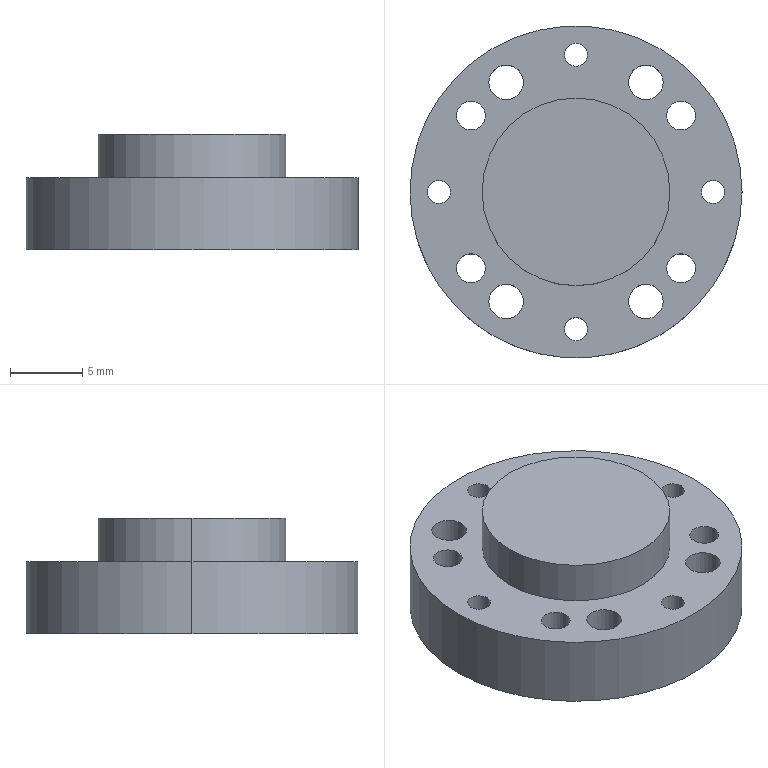CAM job | Mastercam | mm | 1 operations | part box 23 x 23 x 8
1. Drill/Counterbore | 7 - 4 倒角刀